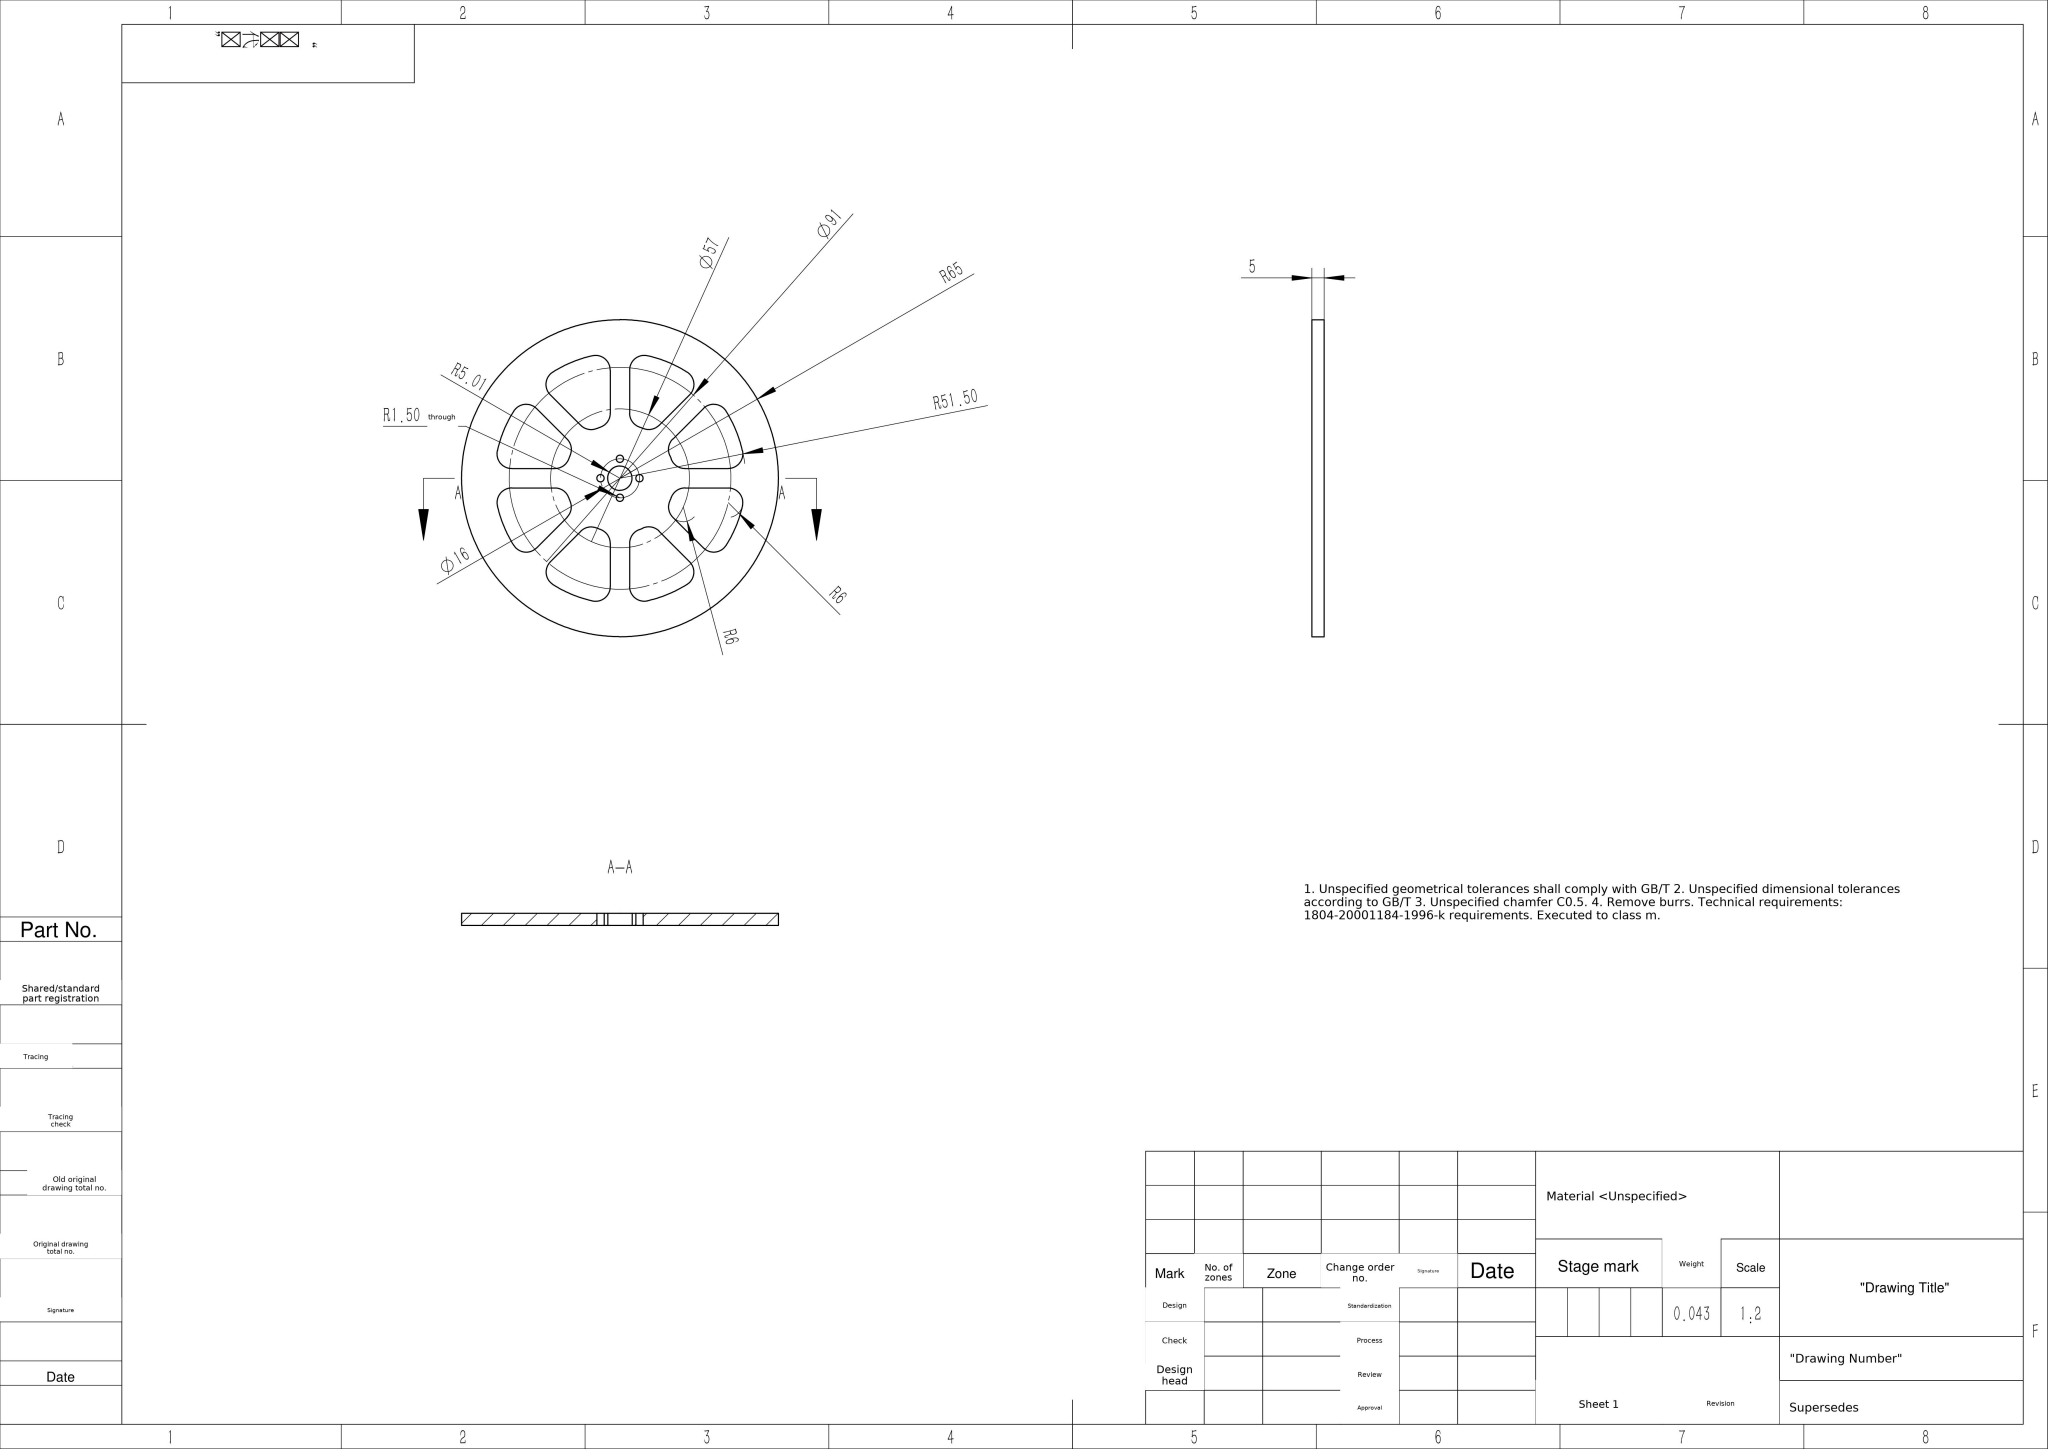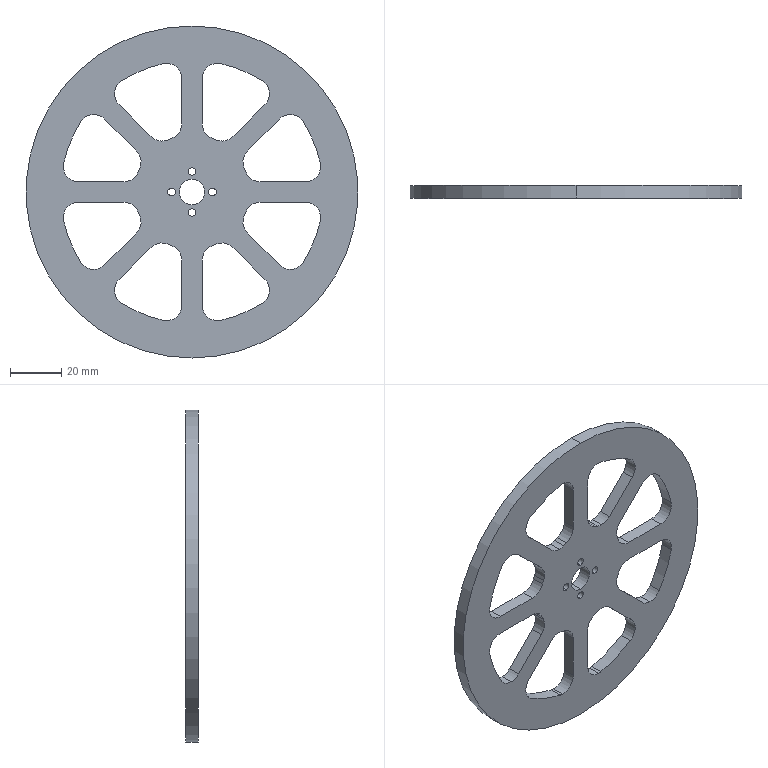Part | SolidWorks | mm | 1 solid | 84 faces | box 130 x 5 x 130 mm | volume 42628 mm3 | cylinder 66 | plane 18 | commonest cylinder face diameters 12 x38 3 x8 45 x8 103 x8 10.01 x2 130 x2